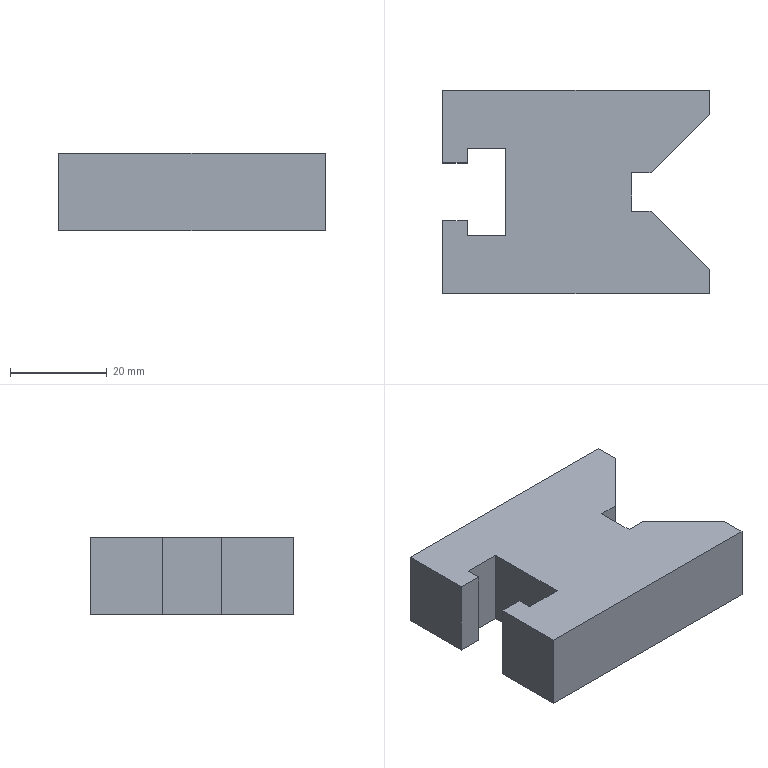Component | NX | V_BLOCK | 1 solid | 20 faces | volume 29344 mm3 | plane 20